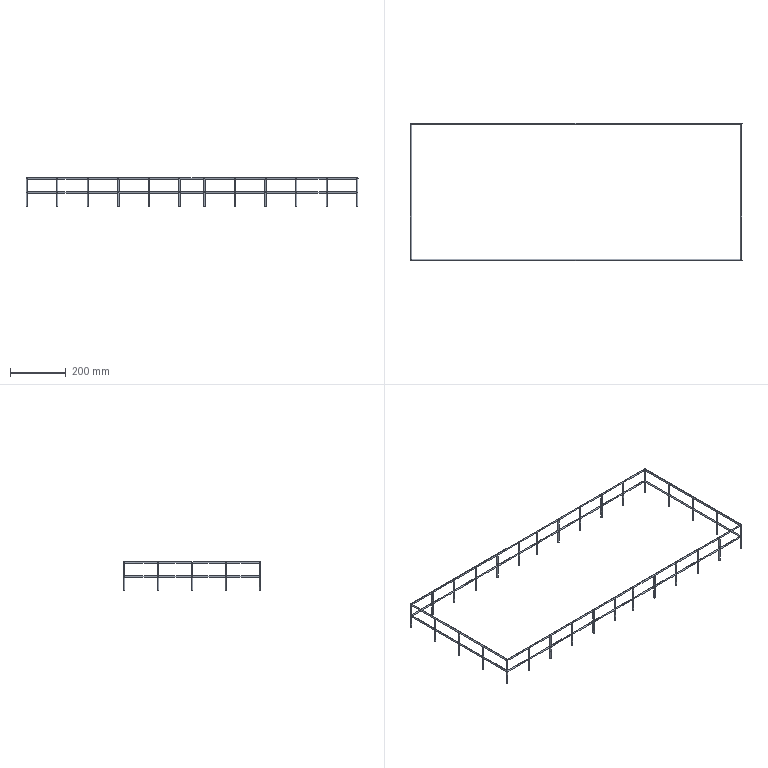Component | SolidWorks | Fence-1 | 1 solid | 226 faces | volume 201661 mm3 | cylinder 172 | plane 54 | commonest cylinder face diameters 5 x164 5.893 x8 | material 304